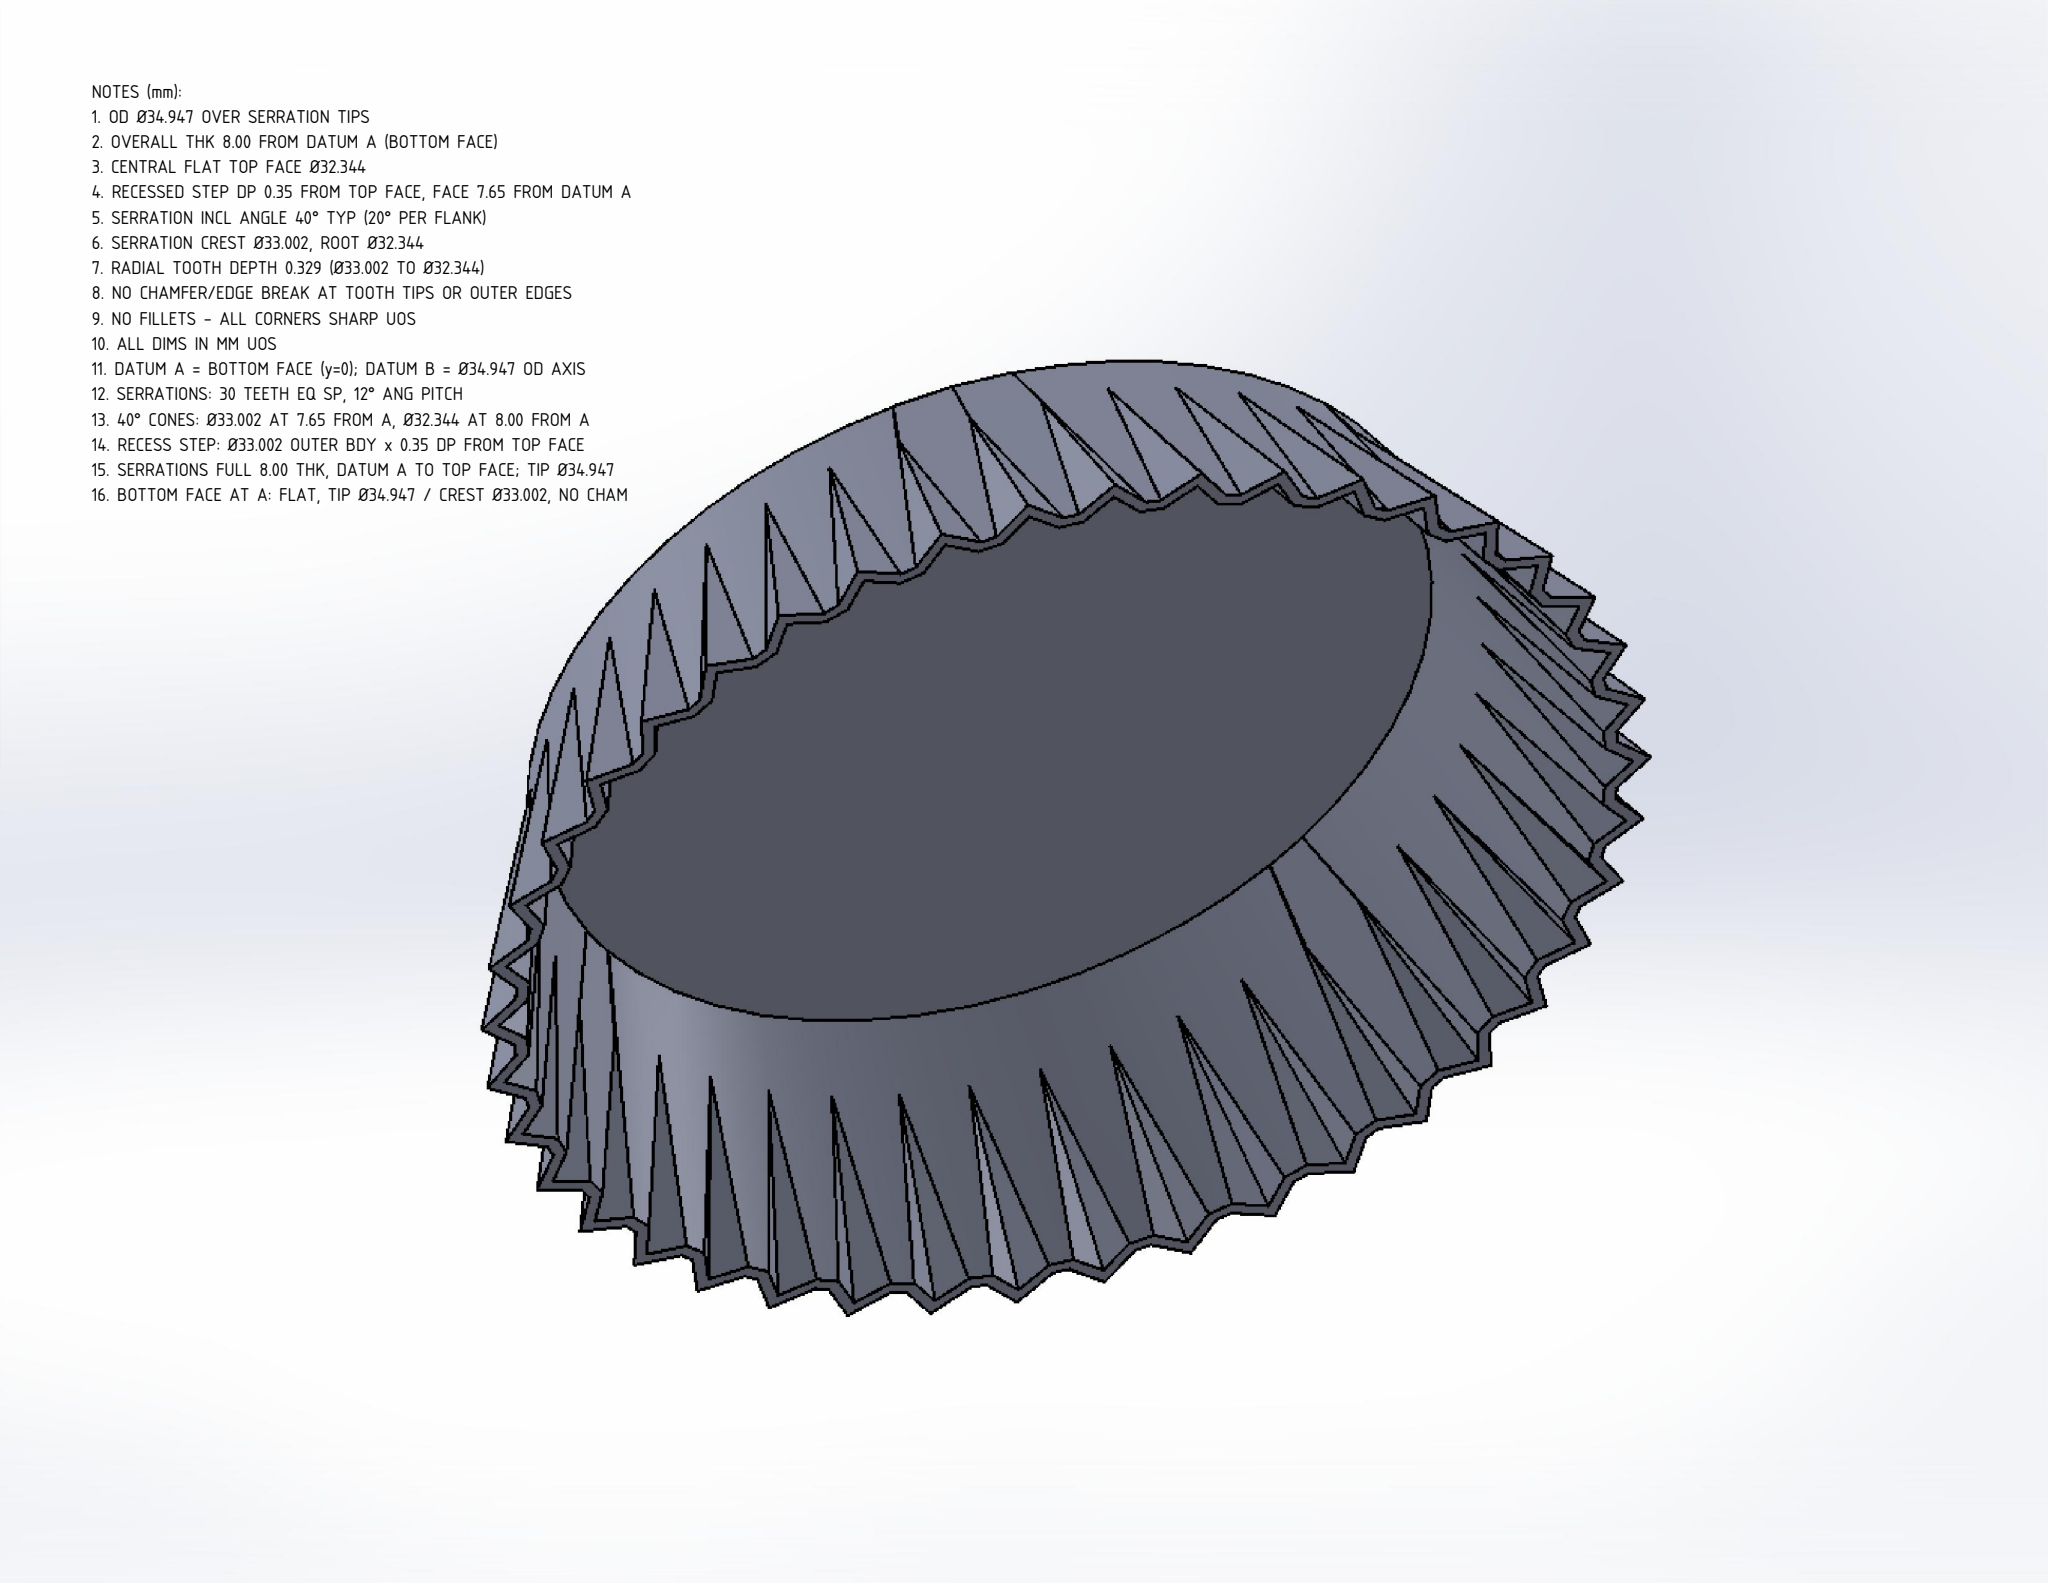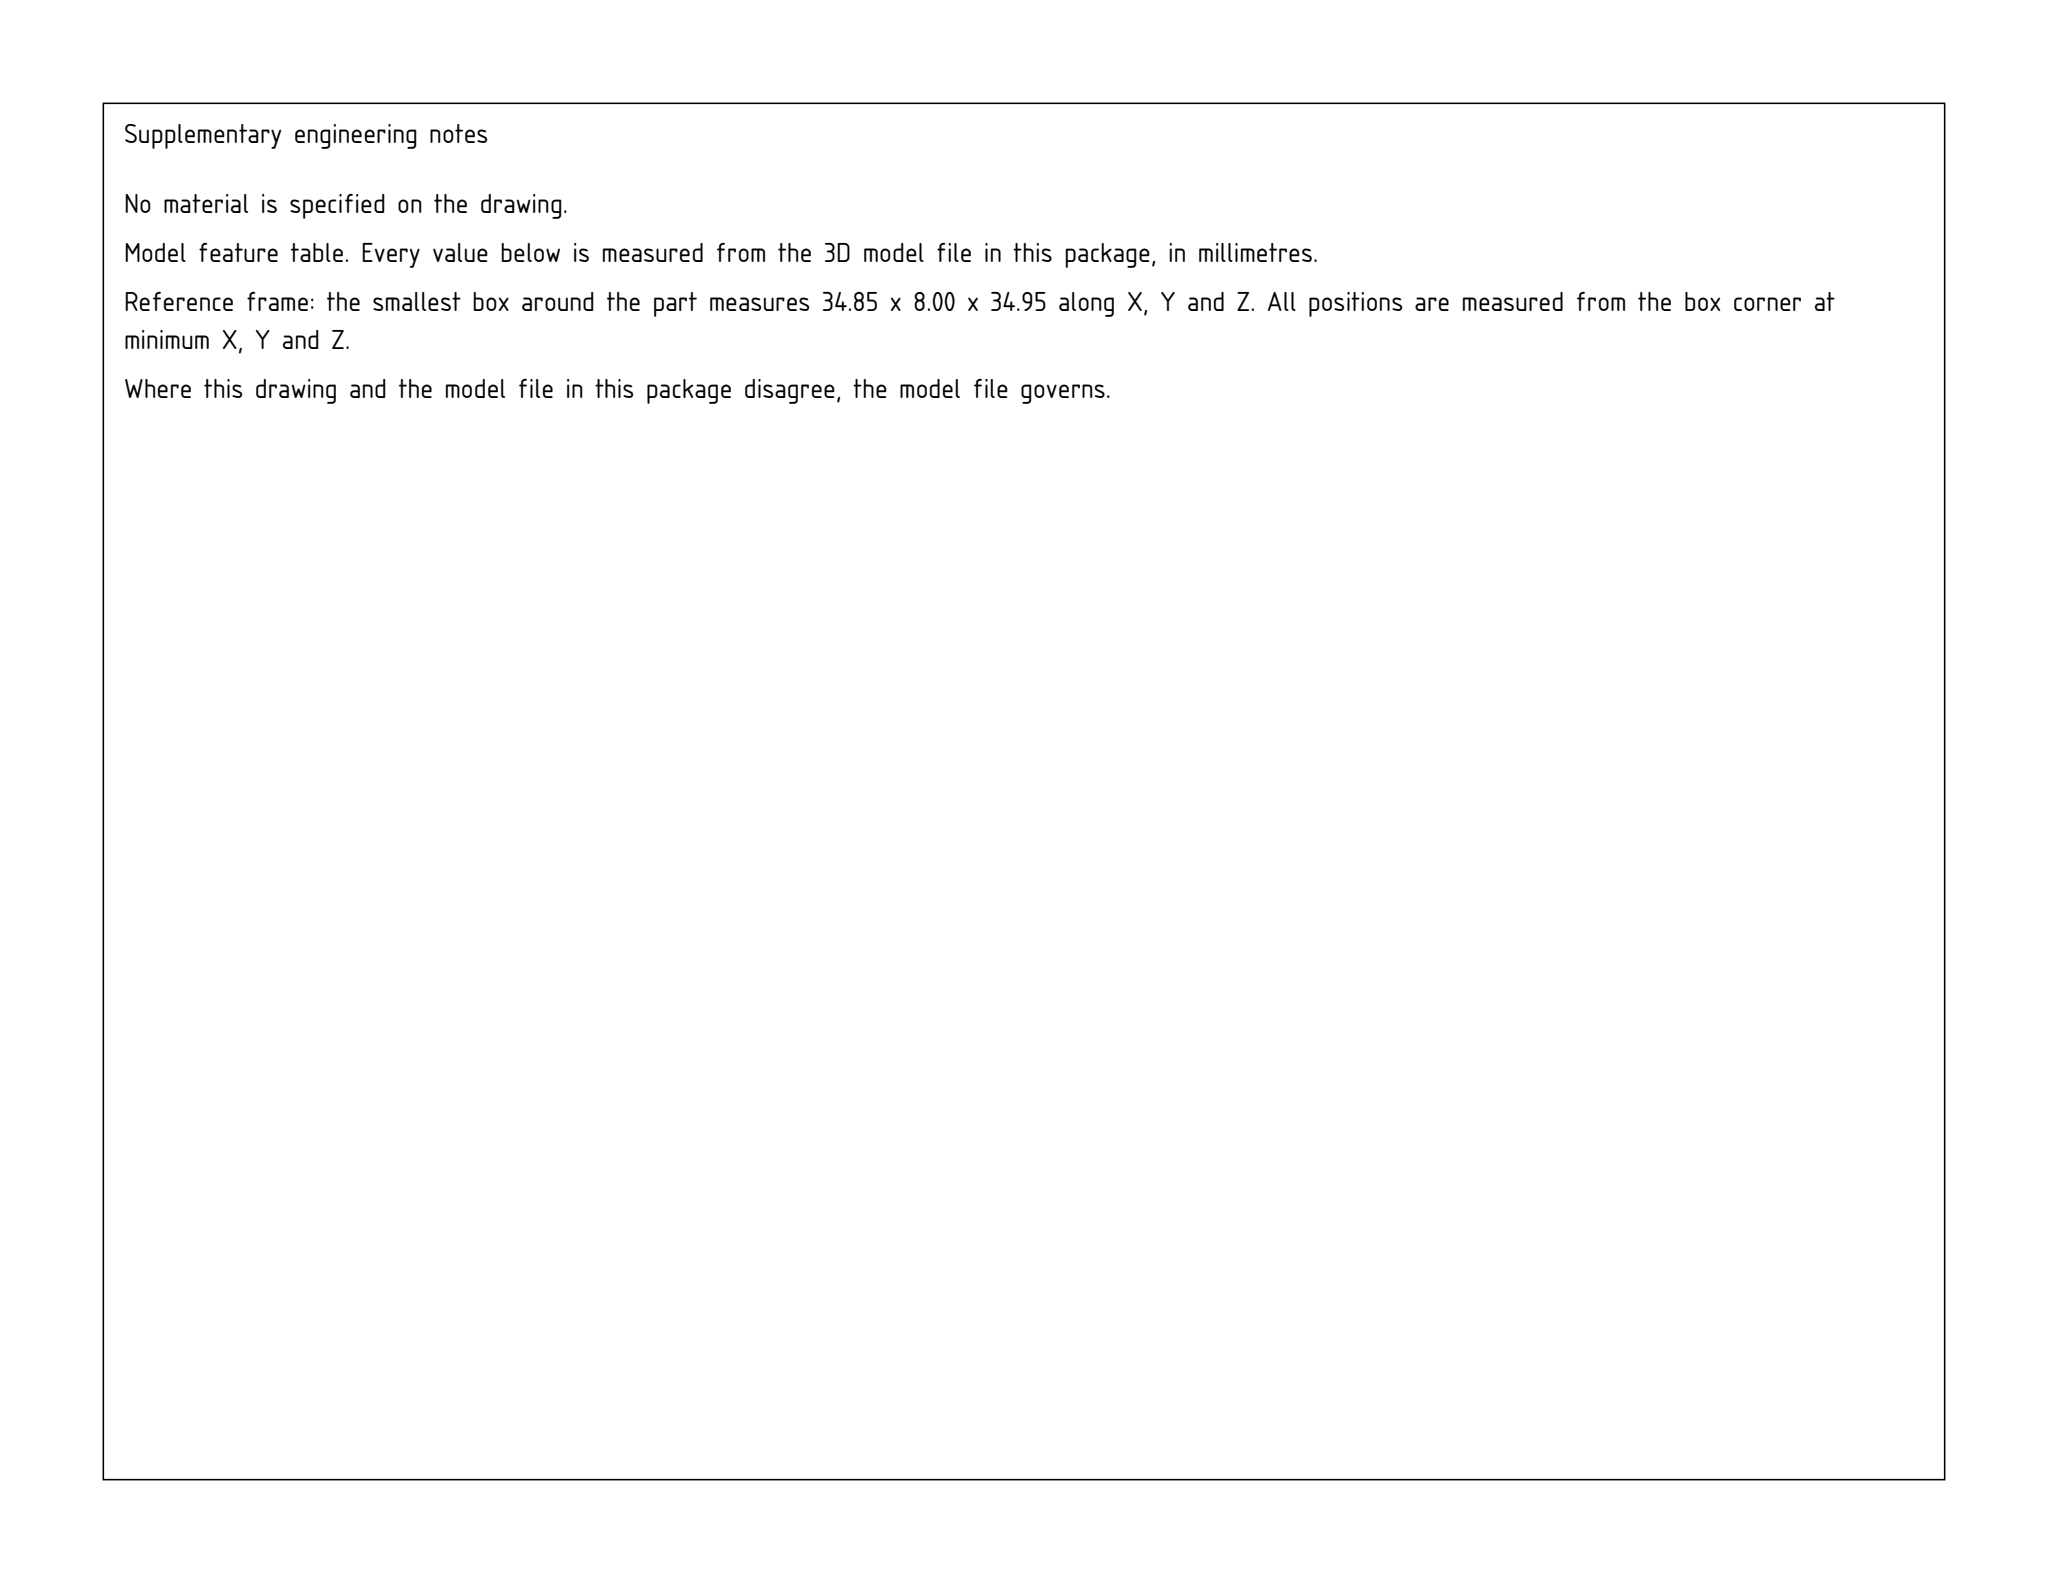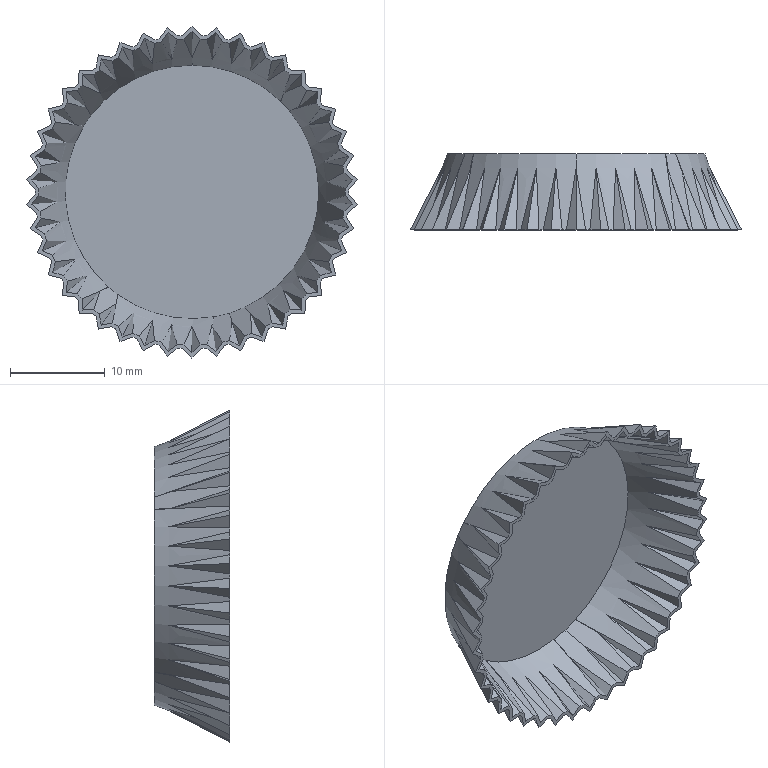Part | SolidWorks | mm | 1 solid | 191 faces | box 34.85 x 8 x 34.95 mm | volume 507 mm3 | plane 181 | cone 10
Drawing notes:
OD Ø34.947 OVER SERRATION TIPS | from the solid: bbox_xyz z = 34.947 (max across tooth tips)
OVERALL THK 8.00 FROM DATUM A (BOTTOM FACE) | from the solid: bbox_xyz y = 8.0; planes y=0 and y=8.0
CENTRAL FLAT TOP FACE Ø32.344 | from the solid: cones ref_dia 32.344 = root/flat face dia; plane y=8.0
RECESSED STEP DP 0.35 FROM TOP FACE, FACE 7.65 FROM DATUM A | from the solid: axis_planes y=7.65 and y=8.0; 8.0-7.65=0.35
SERRATION INCL ANGLE 40° TYP (20° PER FLANK) | from the solid: cones included_angle 40.0 both ref dias
SERRATION CREST Ø33.002, ROOT Ø32.344 | from the solid: cones ref_dia 33.002 and 32.344
RADIAL TOOTH DEPTH 0.329 (Ø33.002 TO Ø32.344) | from the solid: (33.002-32.344)/2 = 0.329
NO CHAMFER/EDGE BREAK AT TOOTH TIPS OR OUTER EDGES | from the solid: no chamfer or conical break faces beyond 40° tooth cones
NO FILLETS - ALL CORNERS SHARP UOS | from the solid: fillet_radii: [] (empty)
ALL DIMS IN MM UOS | from the solid: STEP model units mm, bbox 34.85 x 8.0 x 34.947
DATUM A = BOTTOM FACE (y=0); DATUM B = Ø34.947 OD AXIS | from the solid: axis_planes y=0.0; bbox centered OD 34.947
SERRATIONS: 30 TEETH EQ SP, 12° ANG PITCH | from the solid: BBox 34.947 x 34.85 across flats: 34.85 = 34.947*cos(6°) -> half pitch 6° => 30 teeth
40° CONES: Ø33.002 AT 7.65 FROM A, Ø32.344 AT 8.00 FROM A | from the solid: cones[40.0,33.002] and cones[40.0,32.344]; axis planes y=7.65 and y=8.00, datum A at y=0
RECESS STEP: Ø33.002 OUTER BDY x 0.35 DP FROM TOP FACE | from the solid: planes y=8.00 (top) and y=7.65 -> 0.35 deep; outer ref dia 33.002
SERRATIONS FULL 8.00 THK, DATUM A TO TOP FACE; TIP Ø34.947 | from the solid: bbox_xyz y=8.00 overall, tip OD 34.947; only planes at y=0/7.65/8.00
BOTTOM FACE AT A: FLAT, TIP Ø34.947 / CREST Ø33.002, NO CHAM | from the solid: axis plane y=0.0 (flat), bbox z=34.947, cone ref dia 33.002; fillet_radii empty